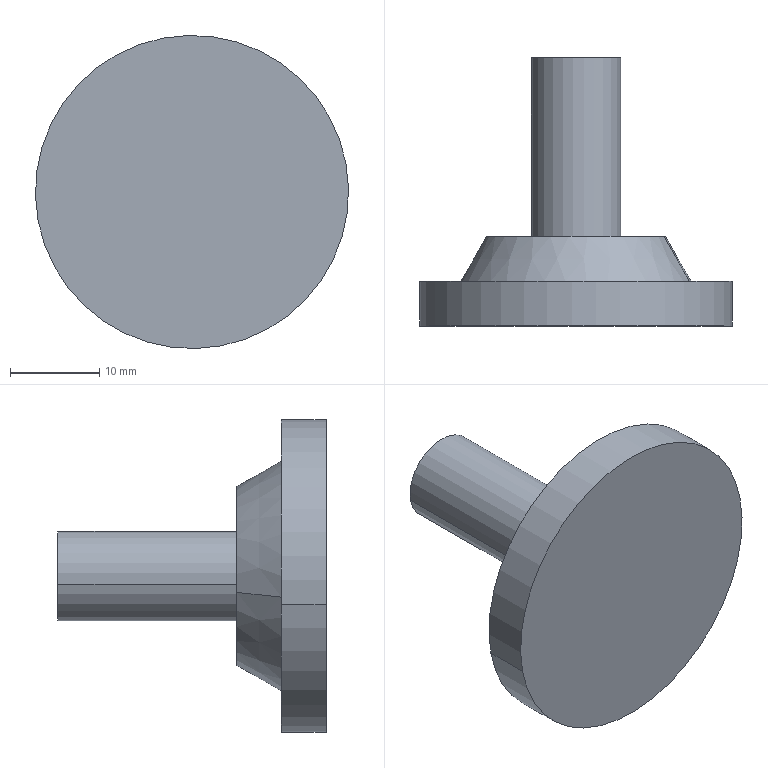Component | SolidWorks | Mirror Part81^Assembly2-12 | 1 solid | 10 faces | box 35 x 30 x 35 mm | volume 8449 mm3 | cylinder 4 | plane 4 | cone 2 | commonest cylinder face diameters 35 x2 10 x2
STEP:
#1=COLOUR_RGB('',0.7922,0.8196,0.9333);
#2=FILL_AREA_STYLE_COLOUR('',#1);
#3=FILL_AREA_STYLE('',(#2));
#4=SURFACE_STYLE_FILL_AREA(#3);
#5=SURFACE_SIDE_STYLE('',(#4));
#6=SURFACE_STYLE_USAGE(.BOTH.,#5);
#7=PRESENTATION_STYLE_ASSIGNMENT((#6));
#8=CARTESIAN_POINT('',(-6.268,-1.102,-86.674));
#9=VERTEX_POINT('',#8);
#10=CARTESIAN_POINT('',(-4.913,-1.102,-86.422));
#11=VERTEX_POINT('',#10);
#12=CARTESIAN_POINT('',(-5.591,-1.102,-86.548));
#13=DIRECTION('',(0.,1.,0.));
#14=DIRECTION('',(0.9831,0.,0.1833));
#15=AXIS2_PLACEMENT_3D('',#12,#13,#14);
#16=CIRCLE('',#15,0.689);
#17=EDGE_CURVE('',#9,#11,#16,.T.);
#18=ORIENTED_EDGE('',*,*,#17,.T.);
#19=CARTESIAN_POINT('',(-4.913,-0.9055,-86.422));
#20=VERTEX_POINT('',#19);
#21=CARTESIAN_POINT('',(-4.913,-1.102,-86.422));
#22=DIRECTION('',(0.,1.,0.));
#23=VECTOR('',#22,39.37);
#24=LINE('',#21,#23);
#25=EDGE_CURVE('',#11,#20,#24,.T.);
#26=ORIENTED_EDGE('',*,*,#25,.T.);
#27=CARTESIAN_POINT('',(-6.268,-0.9055,-86.674));
#28=VERTEX_POINT('',#27);
#29=CARTESIAN_POINT('',(-5.591,-0.9055,-86.548));
#30=DIRECTION('',(0.,1.,0.));
#31=DIRECTION('',(0.9831,0.,0.1833));
#32=AXIS2_PLACEMENT_3D('',#29,#30,#31);
#33=CIRCLE('',#32,0.689);
#34=EDGE_CURVE('',#28,#20,#33,.T.);
#35=ORIENTED_EDGE('',*,*,#34,.F.);
#36=CARTESIAN_POINT('',(-6.268,-1.102,-86.674));
#37=DIRECTION('',(0.,1.,0.));
#38=VECTOR('',#37,39.37);
#39=LINE('',#36,#38);
#40=EDGE_CURVE('',#9,#28,#39,.T.);
#41=ORIENTED_EDGE('',*,*,#40,.F.);
#42=EDGE_LOOP('',(#18,#26,#35,#41));
#43=FACE_OUTER_BOUND('',#42,.T.);
#44=CARTESIAN_POINT('',(-5.591,-1.102,-86.548));
#45=DIRECTION('',(0.,1.,0.));
#46=DIRECTION('',(-0.9831,0.,-0.1833));
#47=AXIS2_PLACEMENT_3D('',#44,#45,#46);
#48=CYLINDRICAL_SURFACE('',#47,0.689);
#49=ADVANCED_FACE('',(#43),#48,.T.);
#50=CARTESIAN_POINT('',(-5.978,-0.7087,-86.62));
#51=VERTEX_POINT('',#50);
#52=CARTESIAN_POINT('',(-5.204,-0.7087,-86.476));
#53=VERTEX_POINT('',#52);
#54=CARTESIAN_POINT('',(-5.591,-0.7087,-86.548));
#55=DIRECTION('',(0.,1.,0.));
#56=DIRECTION('',(0.9831,0.,0.1833));
#57=AXIS2_PLACEMENT_3D('',#54,#55,#56);
#58=CIRCLE('',#57,0.3937);
#59=EDGE_CURVE('',#51,#53,#58,.T.);
#60=ORIENTED_EDGE('',*,*,#59,.F.);
#61=CARTESIAN_POINT('',(-6.089,-0.9055,-86.641));
#62=VERTEX_POINT('',#61);
#63=CARTESIAN_POINT('',(-5.978,-0.7087,-86.62));
#64=DIRECTION('',(-0.4915,-0.866,-0.09163));
#65=VECTOR('',#64,39.37);
#66=LINE('',#63,#65);
#67=EDGE_CURVE('',#51,#62,#66,.T.);
#68=ORIENTED_EDGE('',*,*,#67,.T.);
#69=CARTESIAN_POINT('',(-5.092,-0.9055,-86.455));
#70=VERTEX_POINT('',#69);
#71=CARTESIAN_POINT('',(-5.591,-0.9055,-86.548));
#72=DIRECTION('',(0.,1.,0.));
#73=DIRECTION('',(0.9831,0.,0.1833));
#74=AXIS2_PLACEMENT_3D('',#71,#72,#73);
#75=CIRCLE('',#74,0.5074);
#76=EDGE_CURVE('',#62,#70,#75,.T.);
#77=ORIENTED_EDGE('',*,*,#76,.T.);
#78=CARTESIAN_POINT('',(-5.204,-0.7087,-86.476));
#79=DIRECTION('',(0.4915,-0.866,0.09163));
#80=VECTOR('',#79,39.37);
#81=LINE('',#78,#80);
#82=EDGE_CURVE('',#53,#70,#81,.T.);
#83=ORIENTED_EDGE('',*,*,#82,.F.);
#84=EDGE_LOOP('',(#60,#68,#77,#83));
#85=FACE_OUTER_BOUND('',#84,.T.);
#86=CARTESIAN_POINT('',(-5.591,-0.7087,-86.548));
#87=DIRECTION('',(0.,-1.,0.));
#88=DIRECTION('',(0.9831,0.,0.1833));
#89=AXIS2_PLACEMENT_3D('',#86,#87,#88);
#90=CONICAL_SURFACE('',#89,0.3937,0.5236);
#91=ADVANCED_FACE('',(#85),#90,.T.);
#92=CARTESIAN_POINT('',(-5.397,0.07874,-86.512));
#93=VERTEX_POINT('',#92);
#94=CARTESIAN_POINT('',(-5.784,0.07874,-86.584));
#95=VERTEX_POINT('',#94);
#96=CARTESIAN_POINT('',(-5.591,0.07874,-86.548));
#97=DIRECTION('',(0.,-1.,0.));
#98=DIRECTION('',(-0.9831,0.,-0.1833));
#99=AXIS2_PLACEMENT_3D('',#96,#97,#98);
#100=CIRCLE('',#99,0.1969);
#101=EDGE_CURVE('',#93,#95,#100,.T.);
#102=ORIENTED_EDGE('',*,*,#101,.T.);
#103=CARTESIAN_POINT('',(-5.784,-0.7087,-86.584));
#104=VERTEX_POINT('',#103);
#105=CARTESIAN_POINT('',(-5.784,0.07874,-86.584));
#106=DIRECTION('',(0.,-1.,0.));
#107=VECTOR('',#106,39.37);
#108=LINE('',#105,#107);
#109=EDGE_CURVE('',#95,#104,#108,.T.);
#110=ORIENTED_EDGE('',*,*,#109,.T.);
#111=CARTESIAN_POINT('',(-5.397,-0.7087,-86.512));
#112=VERTEX_POINT('',#111);
#113=CARTESIAN_POINT('',(-5.591,-0.7087,-86.548));
#114=DIRECTION('',(0.,-1.,0.));
#115=DIRECTION('',(-0.9831,0.,-0.1833));
#116=AXIS2_PLACEMENT_3D('',#113,#114,#115);
#117=CIRCLE('',#116,0.1969);
#118=EDGE_CURVE('',#112,#104,#117,.T.);
#119=ORIENTED_EDGE('',*,*,#118,.F.);
#120=CARTESIAN_POINT('',(-5.397,0.07874,-86.512));
#121=DIRECTION('',(0.,-1.,0.));
#122=VECTOR('',#121,39.37);
#123=LINE('',#120,#122);
#124=EDGE_CURVE('',#93,#112,#123,.T.);
#125=ORIENTED_EDGE('',*,*,#124,.F.);
#126=EDGE_LOOP('',(#102,#110,#119,#125));
#127=FACE_OUTER_BOUND('',#126,.T.);
#128=CARTESIAN_POINT('',(-5.591,0.07874,-86.548));
#129=DIRECTION('',(0.,-1.,0.));
#130=DIRECTION('',(0.9831,0.,0.1833));
#131=AXIS2_PLACEMENT_3D('',#128,#129,#130);
#132=CYLINDRICAL_SURFACE('',#131,0.1969);
#133=ADVANCED_FACE('',(#127),#132,.T.);
#134=ORIENTED_EDGE('',*,*,#109,.F.);
#135=CARTESIAN_POINT('',(-5.591,0.07874,-86.548));
#136=DIRECTION('',(0.,-1.,0.));
#137=DIRECTION('',(-0.9831,0.,-0.1833));
#138=AXIS2_PLACEMENT_3D('',#135,#136,#137);
#139=CIRCLE('',#138,0.1969);
#140=EDGE_CURVE('',#95,#93,#139,.T.);
#141=ORIENTED_EDGE('',*,*,#140,.T.);
#142=ORIENTED_EDGE('',*,*,#124,.T.);
#143=CARTESIAN_POINT('',(-5.591,-0.7087,-86.548));
#144=DIRECTION('',(0.,-1.,0.));
#145=DIRECTION('',(-0.9831,0.,-0.1833));
#146=AXIS2_PLACEMENT_3D('',#143,#144,#145);
#147=CIRCLE('',#146,0.1969);
#148=EDGE_CURVE('',#104,#112,#147,.T.);
#149=ORIENTED_EDGE('',*,*,#148,.F.);
#150=EDGE_LOOP('',(#134,#141,#142,#149));
#151=FACE_OUTER_BOUND('',#150,.T.);
#152=CARTESIAN_POINT('',(-5.591,0.07874,-86.548));
#153=DIRECTION('',(0.,-1.,0.));
#154=DIRECTION('',(0.9831,0.,0.1833));
#155=AXIS2_PLACEMENT_3D('',#152,#153,#154);
#156=CYLINDRICAL_SURFACE('',#155,0.1969);
#157=ADVANCED_FACE('',(#151),#156,.T.);
#158=ORIENTED_EDGE('',*,*,#101,.F.);
#159=ORIENTED_EDGE('',*,*,#140,.F.);
#160=EDGE_LOOP('',(#158,#159));
#161=FACE_OUTER_BOUND('',#160,.T.);
#162=CARTESIAN_POINT('',(-5.591,0.07874,-86.548));
#163=DIRECTION('',(0.,1.,0.));
#164=DIRECTION('',(-0.9831,0.,-0.1833));
#165=AXIS2_PLACEMENT_3D('',#162,#163,#164);
#166=PLANE('',#165);
#167=ADVANCED_FACE('',(#161),#166,.T.);
#168=ORIENTED_EDGE('',*,*,#67,.F.);
#169=CARTESIAN_POINT('',(-5.591,-0.7087,-86.548));
#170=DIRECTION('',(0.,1.,0.));
#171=DIRECTION('',(0.9831,0.,0.1833));
#172=AXIS2_PLACEMENT_3D('',#169,#170,#171);
#173=CIRCLE('',#172,0.3937);
#174=EDGE_CURVE('',#53,#51,#173,.T.);
#175=ORIENTED_EDGE('',*,*,#174,.F.);
#176=ORIENTED_EDGE('',*,*,#82,.T.);
#177=CARTESIAN_POINT('',(-5.591,-0.9055,-86.548));
#178=DIRECTION('',(0.,1.,0.));
#179=DIRECTION('',(0.9831,0.,0.1833));
#180=AXIS2_PLACEMENT_3D('',#177,#178,#179);
#181=CIRCLE('',#180,0.5074);
#182=EDGE_CURVE('',#70,#62,#181,.T.);
#183=ORIENTED_EDGE('',*,*,#182,.T.);
#184=EDGE_LOOP('',(#168,#175,#176,#183));
#185=FACE_OUTER_BOUND('',#184,.T.);
#186=CARTESIAN_POINT('',(-5.591,-0.7087,-86.548));
#187=DIRECTION('',(0.,-1.,0.));
#188=DIRECTION('',(0.9831,0.,0.1833));
#189=AXIS2_PLACEMENT_3D('',#186,#187,#188);
#190=CONICAL_SURFACE('',#189,0.3937,0.5236);
#191=ADVANCED_FACE('',(#185),#190,.T.);
#192=ORIENTED_EDGE('',*,*,#118,.T.);
#193=ORIENTED_EDGE('',*,*,#148,.T.);
#194=EDGE_LOOP('',(#192,#193));
#195=FACE_BOUND('',#194,.T.);
#196=ORIENTED_EDGE('',*,*,#174,.T.);
#197=ORIENTED_EDGE('',*,*,#59,.T.);
#198=EDGE_LOOP('',(#196,#197));
#199=FACE_OUTER_BOUND('',#198,.T.);
#200=CARTESIAN_POINT('',(-5.591,-0.7087,-86.548));
#201=DIRECTION('',(0.,-1.,0.));
#202=DIRECTION('',(0.9831,0.,0.1833));
#203=AXIS2_PLACEMENT_3D('',#200,#201,#202);
#204=PLANE('',#203);
#205=ADVANCED_FACE('',(#195,#199),#204,.F.);
#206=ORIENTED_EDGE('',*,*,#25,.F.);
#207=CARTESIAN_POINT('',(-5.591,-1.102,-86.548));
#208=DIRECTION('',(0.,1.,0.));
#209=DIRECTION('',(0.9831,0.,0.1833));
#210=AXIS2_PLACEMENT_3D('',#207,#208,#209);
#211=CIRCLE('',#210,0.689);
#212=EDGE_CURVE('',#11,#9,#211,.T.);
#213=ORIENTED_EDGE('',*,*,#212,.T.);
#214=ORIENTED_EDGE('',*,*,#40,.T.);
#215=CARTESIAN_POINT('',(-5.591,-0.9055,-86.548));
#216=DIRECTION('',(0.,1.,0.));
#217=DIRECTION('',(0.9831,0.,0.1833));
#218=AXIS2_PLACEMENT_3D('',#215,#216,#217);
#219=CIRCLE('',#218,0.689);
#220=EDGE_CURVE('',#20,#28,#219,.T.);
#221=ORIENTED_EDGE('',*,*,#220,.F.);
#222=EDGE_LOOP('',(#206,#213,#214,#221));
#223=FACE_OUTER_BOUND('',#222,.T.);
#224=CARTESIAN_POINT('',(-5.591,-1.102,-86.548));
#225=DIRECTION('',(0.,1.,0.));
#226=DIRECTION('',(-0.9831,0.,-0.1833));
#227=AXIS2_PLACEMENT_3D('',#224,#225,#226);
#228=CYLINDRICAL_SURFACE('',#227,0.689);
#229=ADVANCED_FACE('',(#223),#228,.T.);
#230=ORIENTED_EDGE('',*,*,#17,.F.);
#231=ORIENTED_EDGE('',*,*,#212,.F.);
#232=EDGE_LOOP('',(#230,#231));
#233=FACE_OUTER_BOUND('',#232,.T.);
#234=CARTESIAN_POINT('',(-5.591,-1.102,-86.548));
#235=DIRECTION('',(0.,-1.,0.));
#236=DIRECTION('',(0.9831,0.,0.1833));
#237=AXIS2_PLACEMENT_3D('',#234,#235,#236);
#238=PLANE('',#237);
#239=ADVANCED_FACE('',(#233),#238,.T.);
#240=ORIENTED_EDGE('',*,*,#182,.F.);
#241=ORIENTED_EDGE('',*,*,#76,.F.);
#242=EDGE_LOOP('',(#240,#241));
#243=FACE_BOUND('',#242,.T.);
#244=ORIENTED_EDGE('',*,*,#34,.T.);
#245=ORIENTED_EDGE('',*,*,#220,.T.);
#246=EDGE_LOOP('',(#244,#245));
#247=FACE_OUTER_BOUND('',#246,.T.);
#248=CARTESIAN_POINT('',(-5.591,-0.9055,-86.548));
#249=DIRECTION('',(0.,-1.,0.));
#250=DIRECTION('',(0.9831,0.,0.1833));
#251=AXIS2_PLACEMENT_3D('',#248,#249,#250);
#252=PLANE('',#251);
#253=ADVANCED_FACE('',(#243,#247),#252,.F.);
#254=CLOSED_SHELL('',(#49,#91,#133,#157,#167,#191,#205,#229,#239,#253));
#255=MANIFOLD_SOLID_BREP('',#254);
#256=STYLED_ITEM('',(#7),#255);
#257=PRESENTATION_LAYER_ASSIGNMENT('','',(#256));
#258=(LENGTH_UNIT()NAMED_UNIT(*)SI_UNIT($,.METRE.));
#259=LENGTH_MEASURE_WITH_UNIT(LENGTH_MEASURE(0.0254),#258);
#260=DIMENSIONAL_EXPONENTS(1.,0.,0.,0.,0.,0.,0.);
#261=(CONVERSION_BASED_UNIT('',#259)LENGTH_UNIT()NAMED_UNIT(#260));
#262=UNCERTAINTY_MEASURE_WITH_UNIT(LENGTH_MEASURE(0.00001),#261,'','');
#263=(NAMED_UNIT(*)PLANE_ANGLE_UNIT()SI_UNIT($,.RADIAN.));
#264=(NAMED_UNIT(*)SI_UNIT($,.STERADIAN.)SOLID_ANGLE_UNIT());
#265=(GEOMETRIC_REPRESENTATION_CONTEXT(3)GLOBAL_UNCERTAINTY_ASSIGNED_CONTEXT((#262))GLOBAL_UNIT_ASSIGNED_CONTEXT((#261,#263,#264))REPRESENTATION_CONTEXT('',''));
#266=MECHANICAL_DESIGN_GEOMETRIC_PRESENTATION_REPRESENTATION('',(#256),#265);
#267=CARTESIAN_POINT('',(0.,0.,0.));
#268=DIRECTION('',(0.,0.,1.));
#269=DIRECTION('',(1.,0.,0.));
#270=AXIS2_PLACEMENT_3D('',#267,#268,#269);
#271=(LENGTH_UNIT()NAMED_UNIT(*)SI_UNIT($,.METRE.));
#272=LENGTH_MEASURE_WITH_UNIT(LENGTH_MEASURE(0.0254),#271);
#273=DIMENSIONAL_EXPONENTS(1.,0.,0.,0.,0.,0.,0.);
#274=(CONVERSION_BASED_UNIT('',#272)LENGTH_UNIT()NAMED_UNIT(#273));
#275=UNCERTAINTY_MEASURE_WITH_UNIT(LENGTH_MEASURE(0.00001),#274,'','');
#276=(NAMED_UNIT(*)PLANE_ANGLE_UNIT()SI_UNIT($,.RADIAN.));
#277=(NAMED_UNIT(*)SI_UNIT($,.STERADIAN.)SOLID_ANGLE_UNIT());
#278=(GEOMETRIC_REPRESENTATION_CONTEXT(3)GLOBAL_UNCERTAINTY_ASSIGNED_CONTEXT((#275))GLOBAL_UNIT_ASSIGNED_CONTEXT((#274,#276,#277))REPRESENTATION_CONTEXT('',''));
#279=ADVANCED_BREP_SHAPE_REPRESENTATION('',(#255,#270),#278);